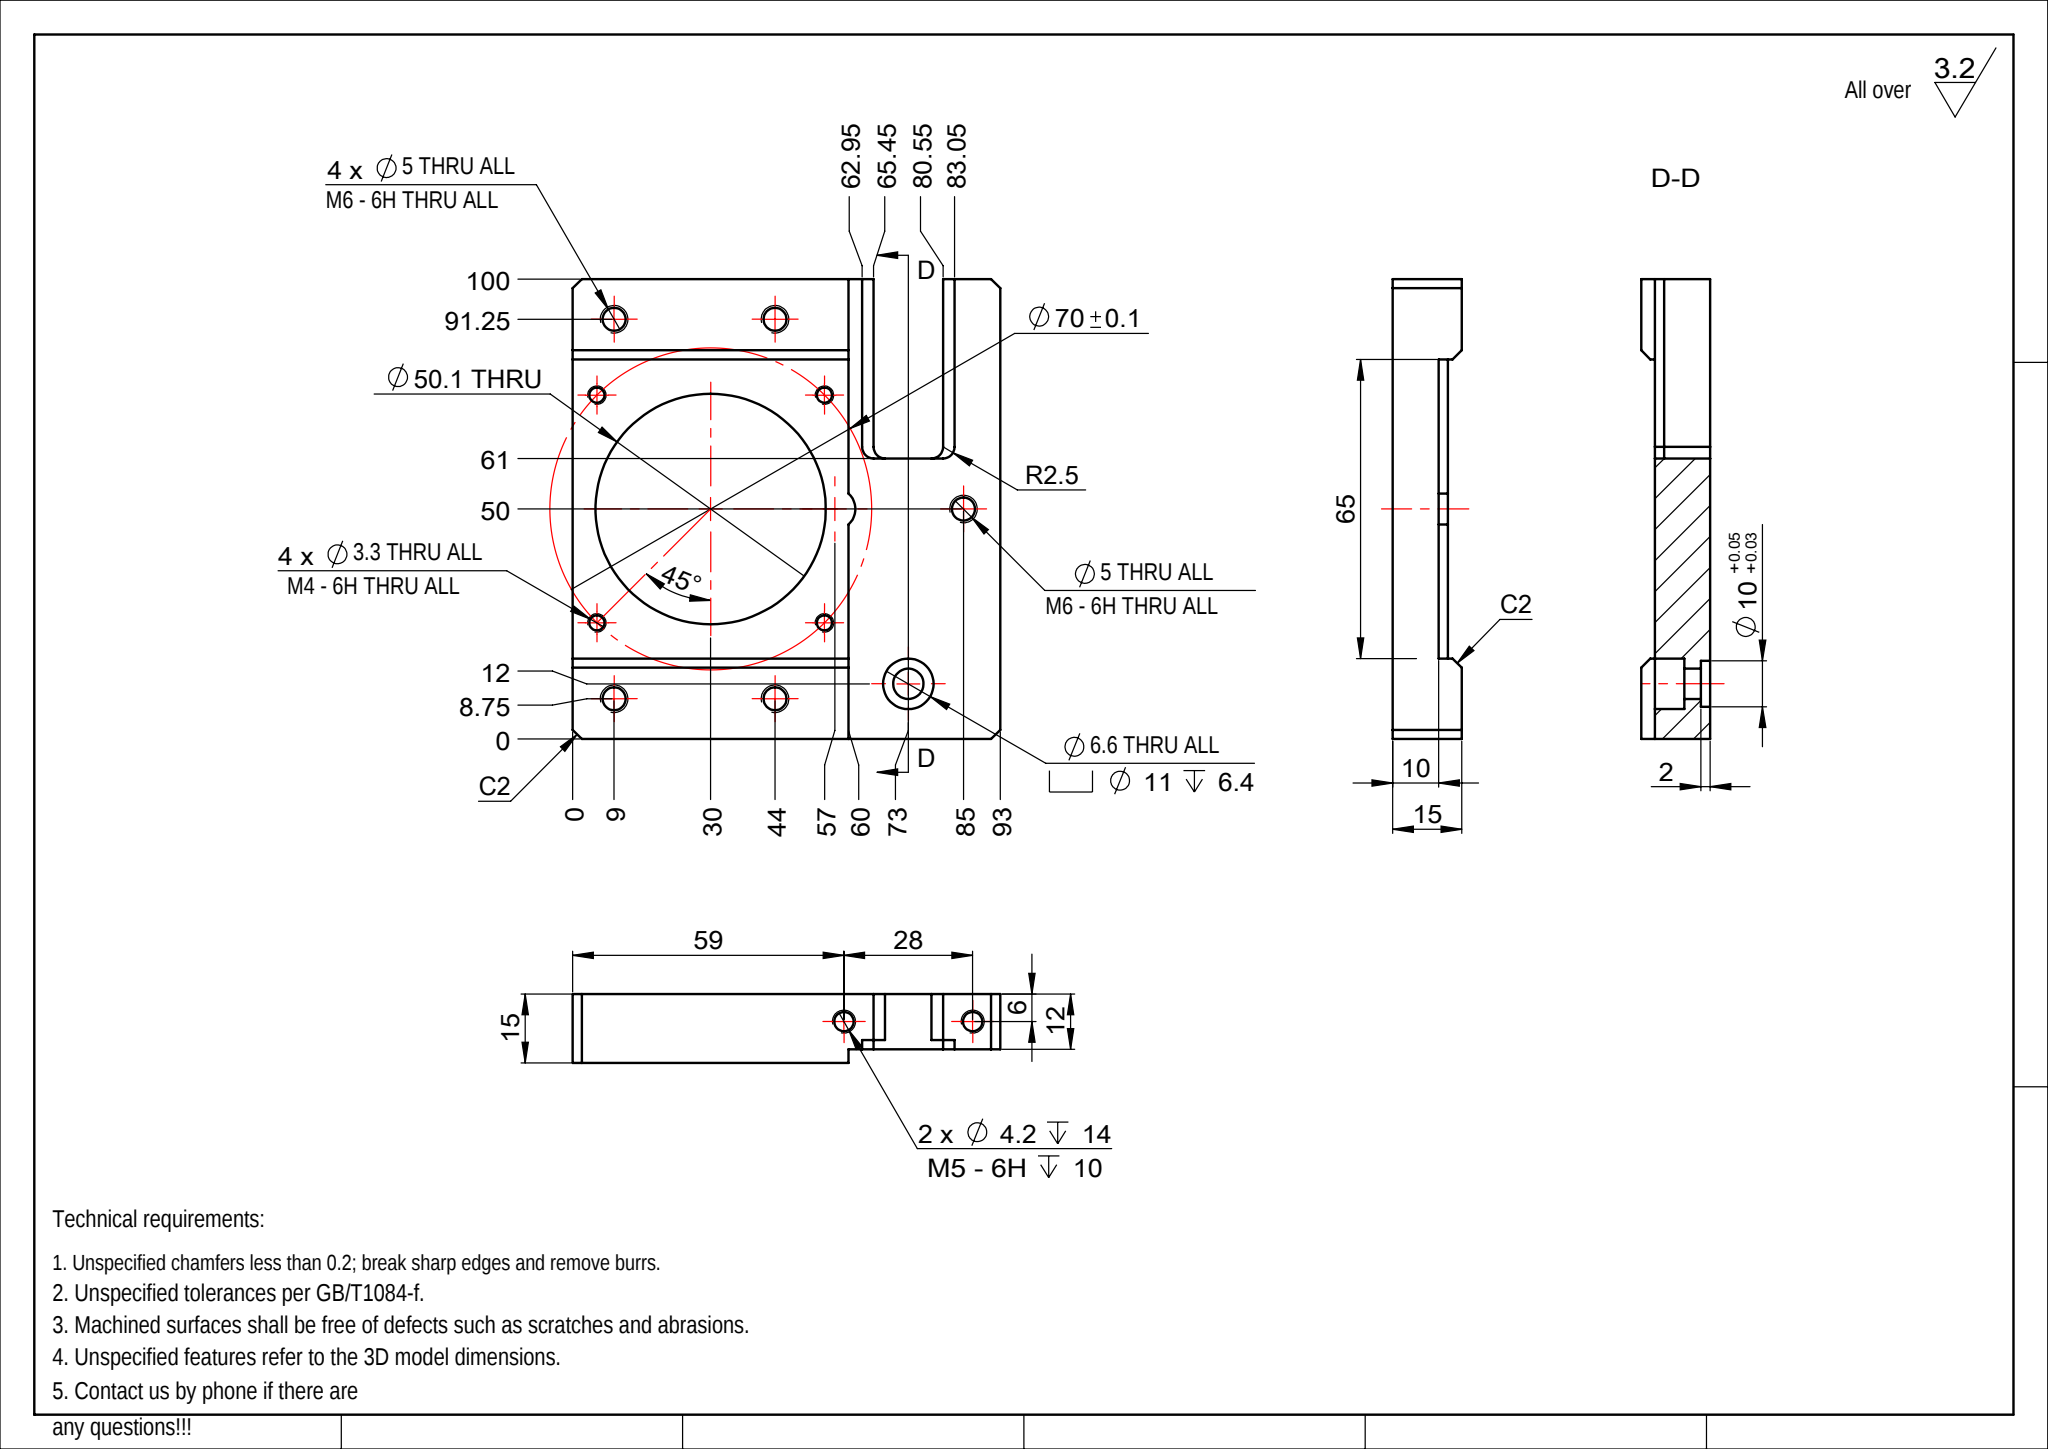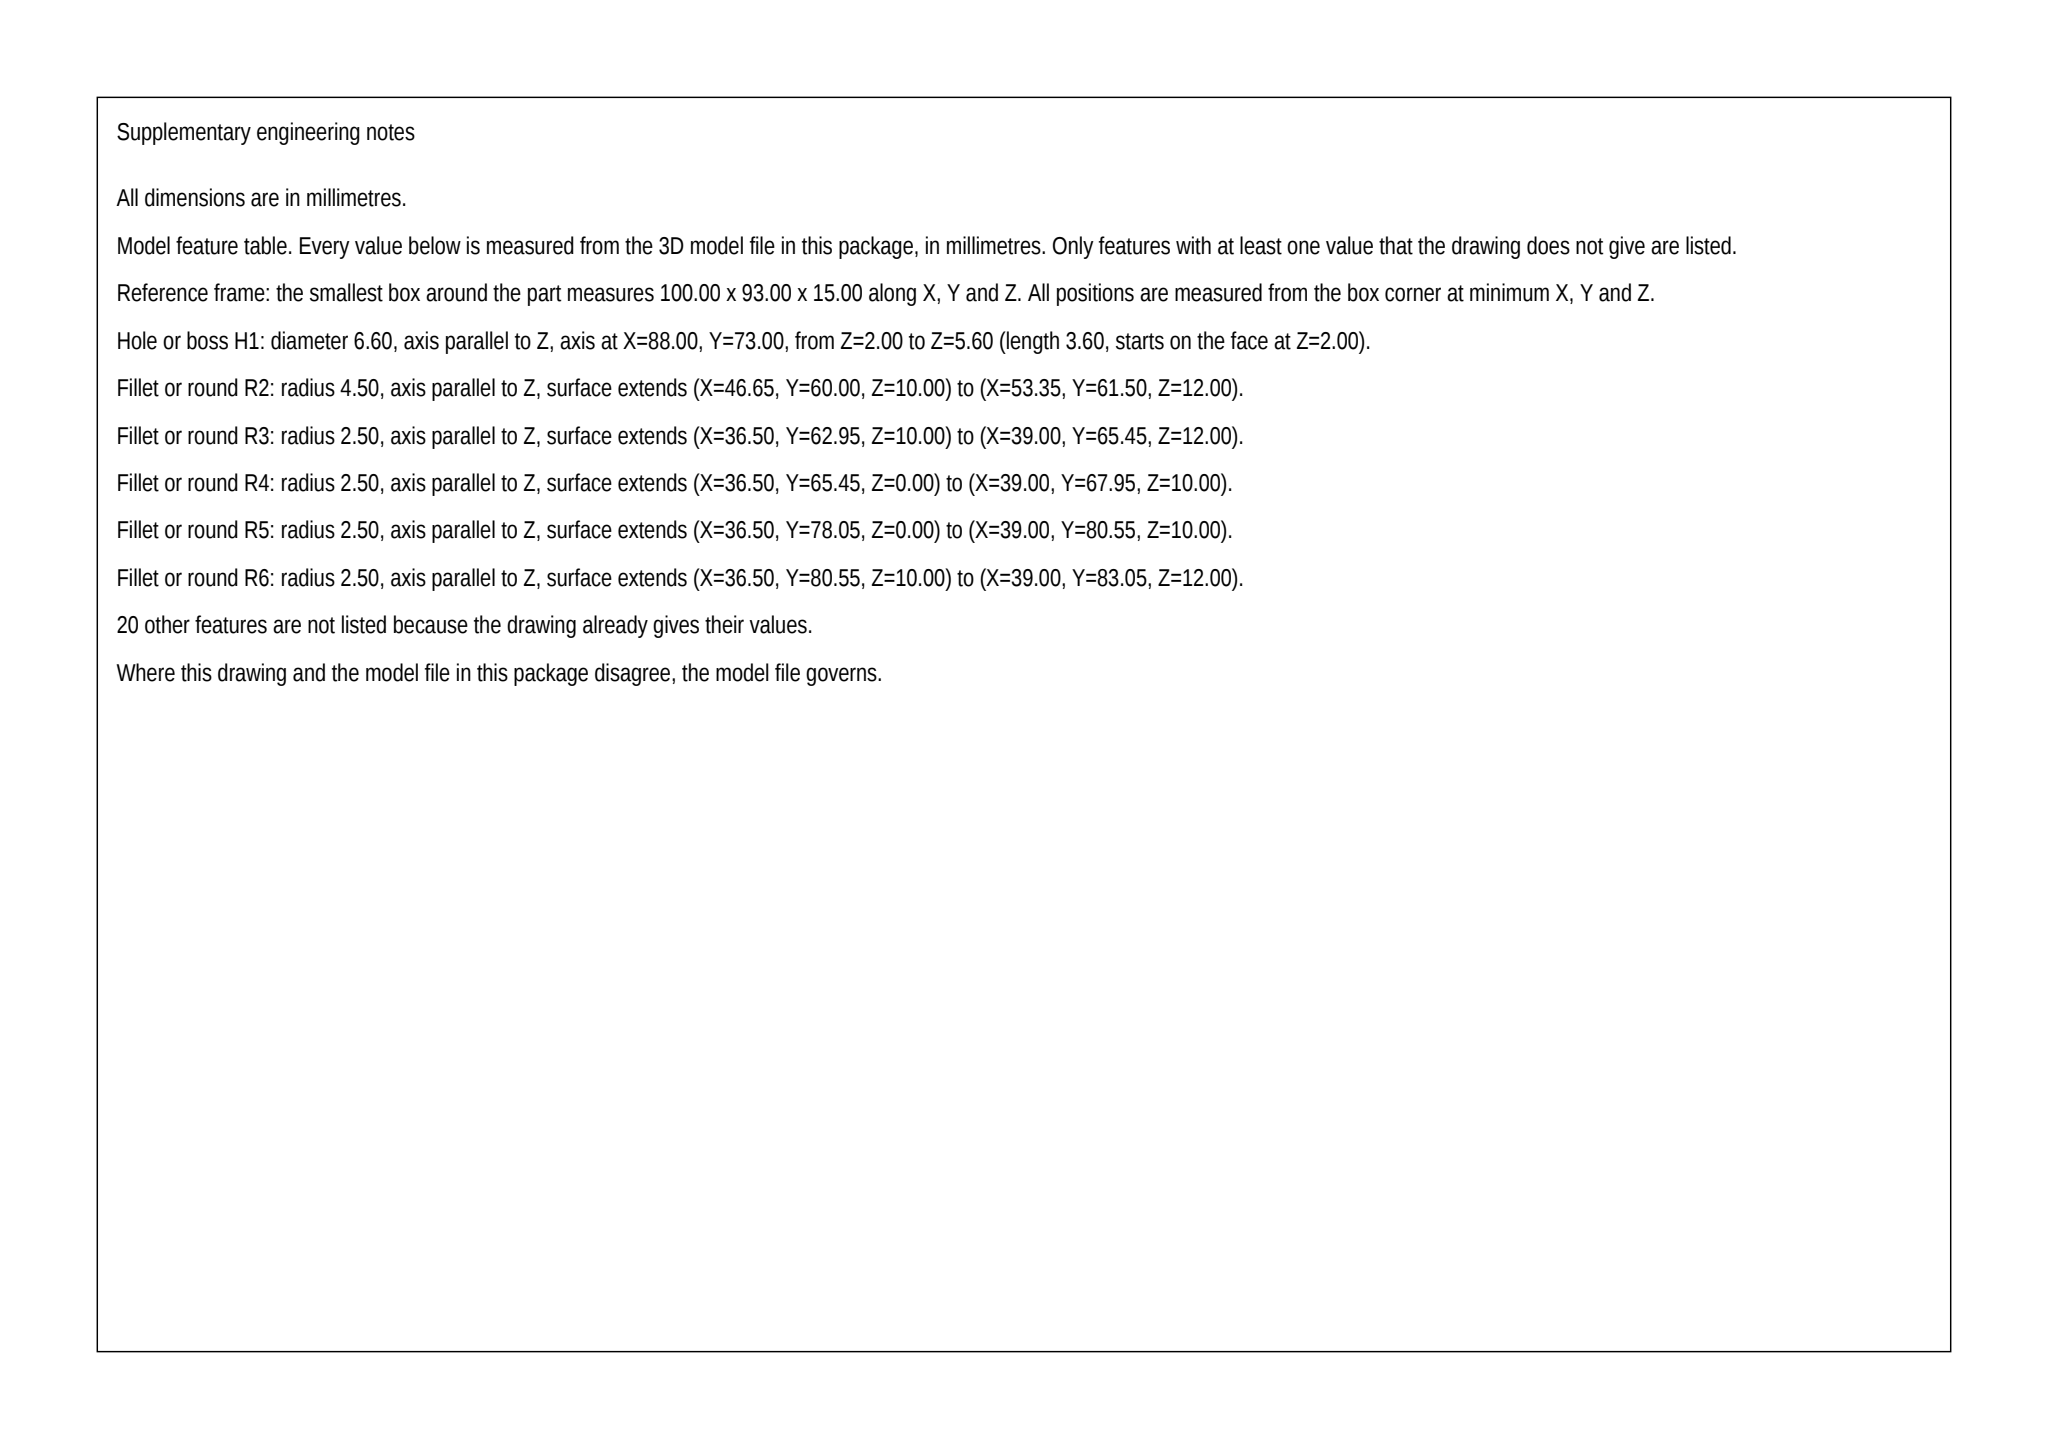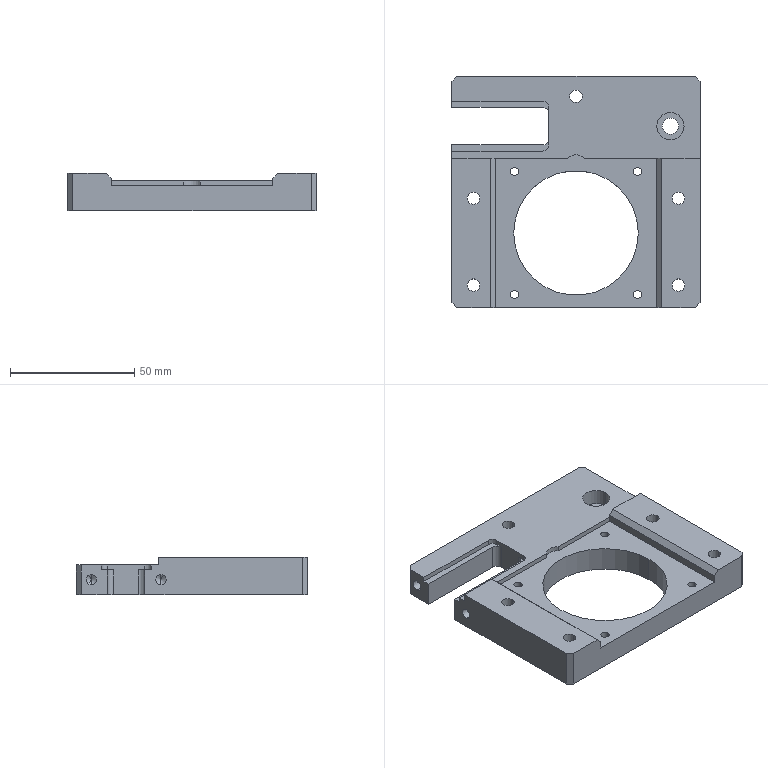Part | SolidWorks | mm | 1 solid | 70 faces | box 100 x 93 x 15 mm | volume 79556 mm3 | cylinder 35 | plane 31 | cone 4 | commonest cylinder face diameters 5 x14 3.3 x8 4.2 x4 11 x2 6.6 x2 10 x2 50.1 x2 9 x1